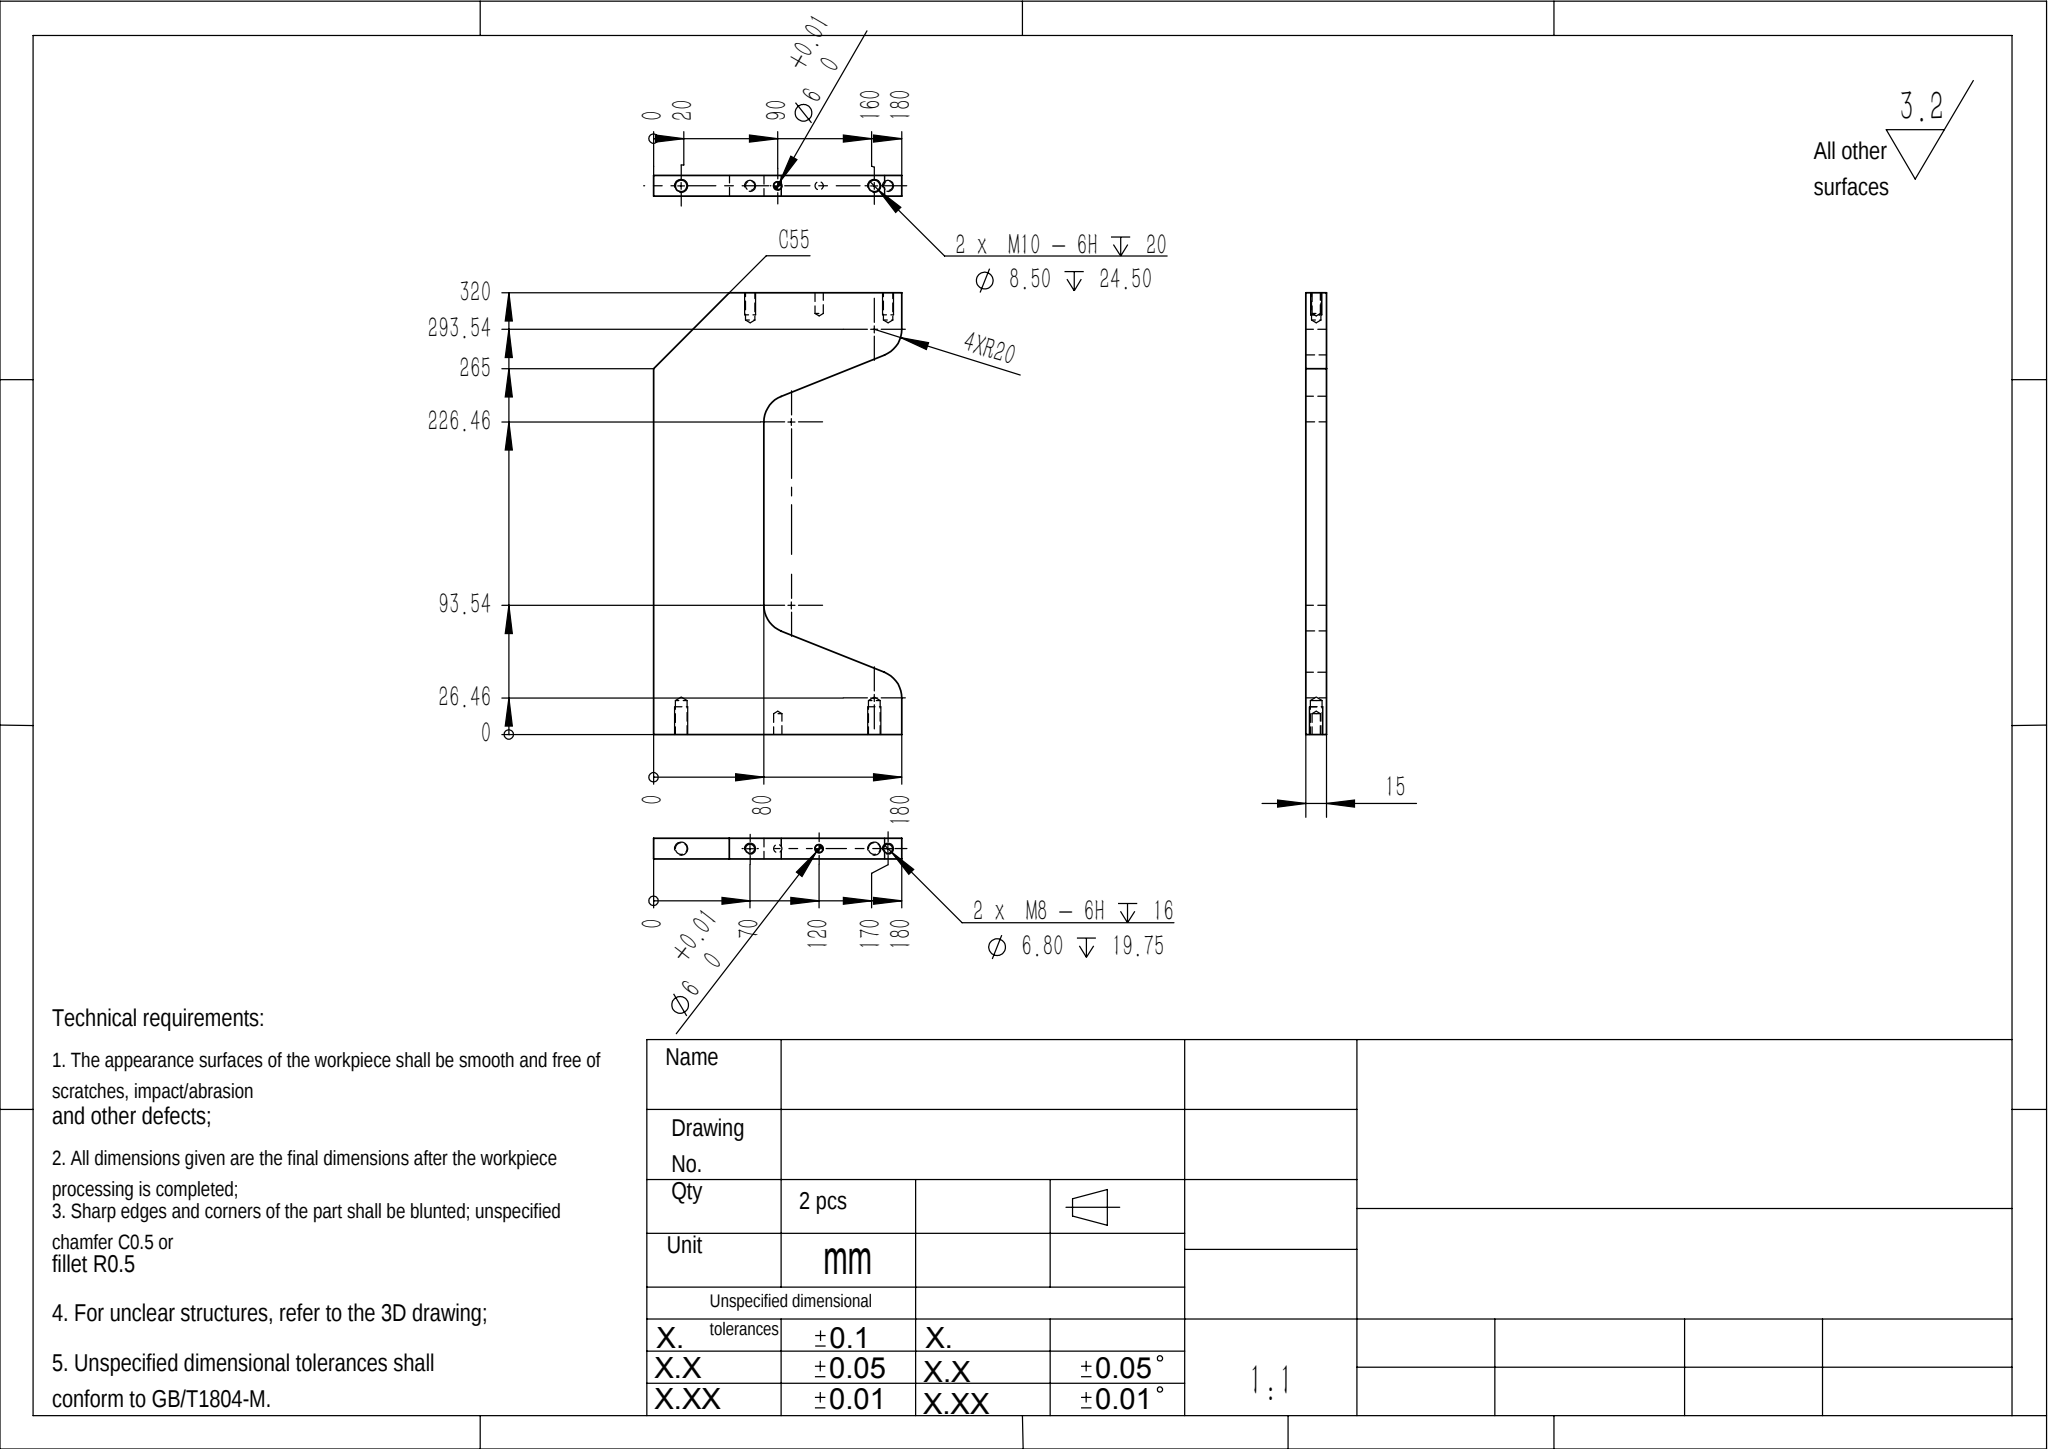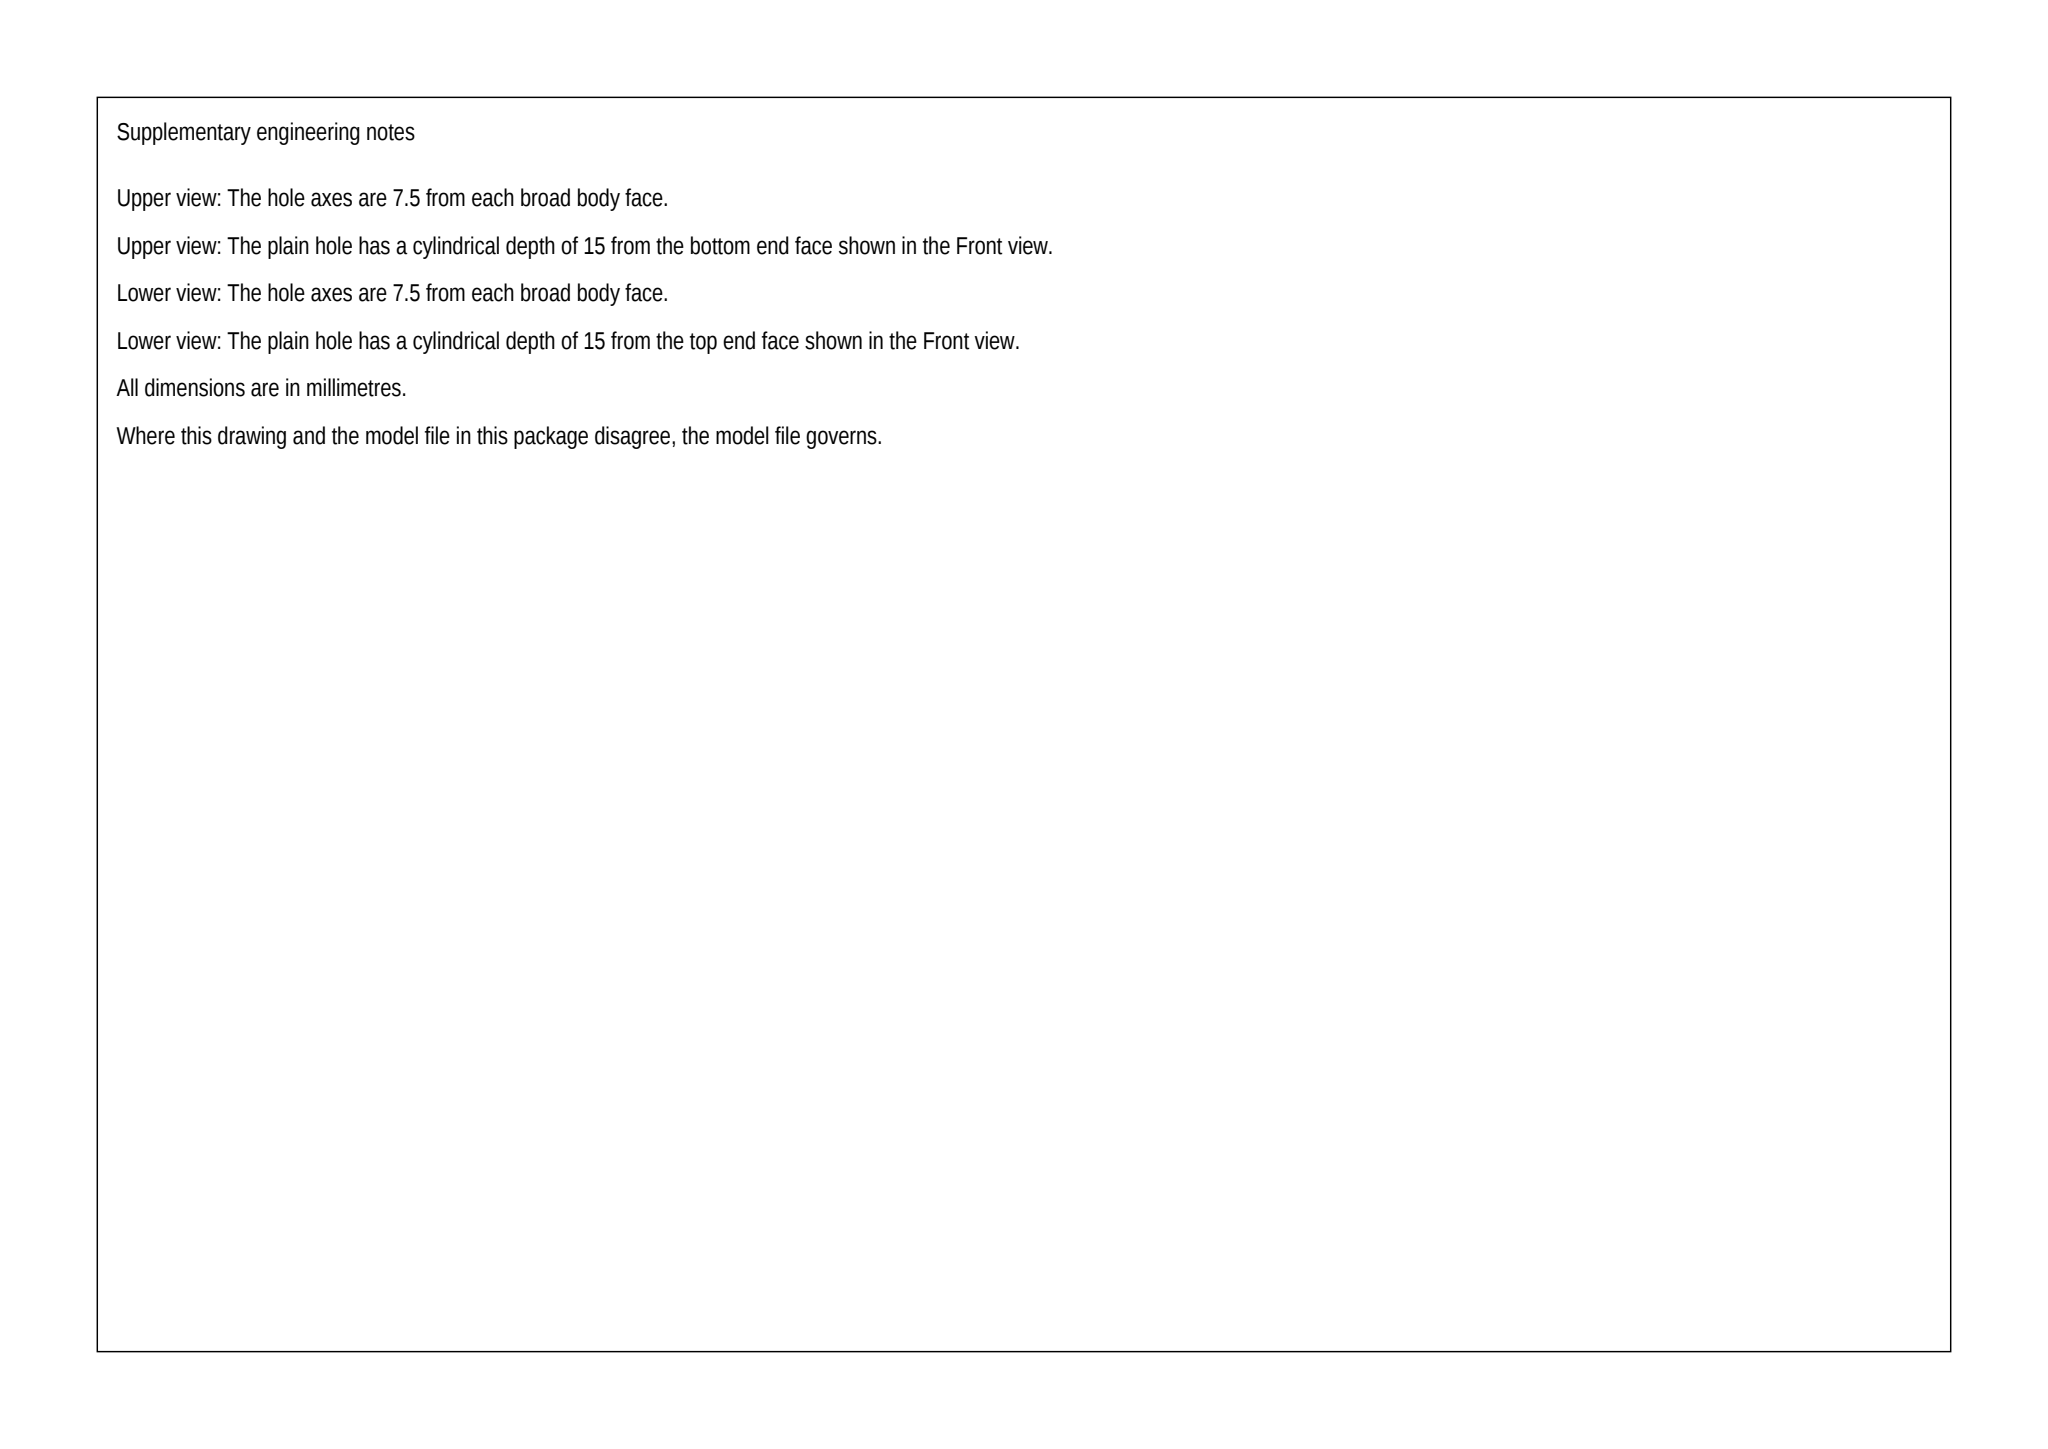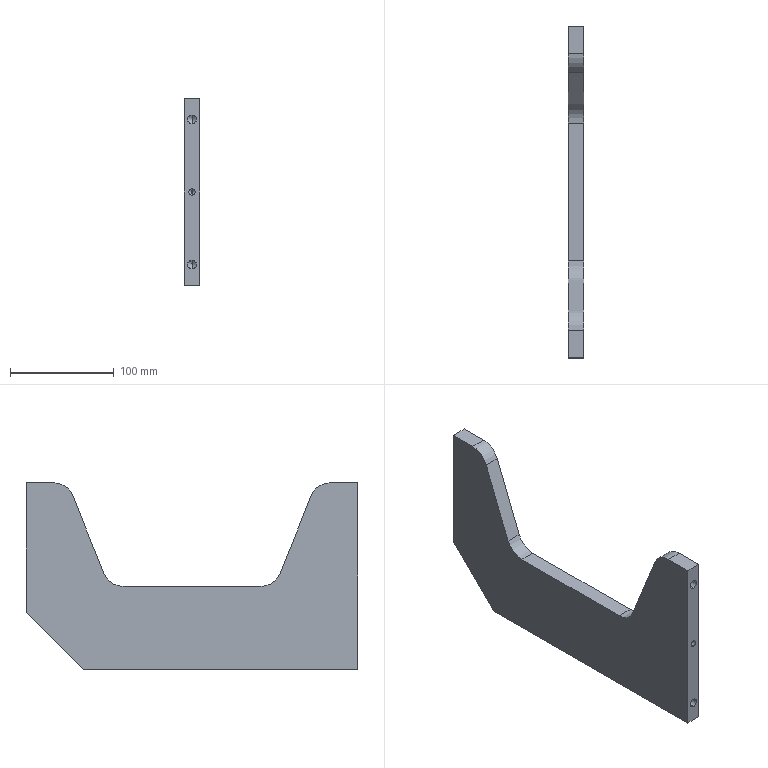Part | SolidWorks | mm | material C55 | 1 solid | 39 faces | box 15 x 320 x 180 mm | volume 536069 mm3 | cylinder 16 | cone 12 | plane 11 | commonest cylinder face diameters 6 x4 8.5 x4 6.8 x4 40 x4
build123d program:
from build123d import *

# Parameters (mm, degrees)
BOSS_EXTRUDE1_DEPTH            = 15
CHAMFER1_SIZE                  = 55
M8_TAPPED_HOLE2_D              = 6.8
M8_TAPPED_HOLE2_DEPTH          = 19.75
M8_TAPPED_HOLE2_TIP            = 2.043
M10_TAPPED_HOLE4_D             = 8.5
M10_TAPPED_HOLE4_DEPTH         = 24.5
M10_TAPPED_HOLE4_TIP           = 2.554
FILLET1_R                      = 20
SIZE_MM_DOWEL_PIN_HOLE_1_D     = 6
SIZE_MM_DOWEL_PIN_HOLE_1_DEPTH = 15
SIZE_MM_DOWEL_PIN_HOLE_1_TIP   = 1.803
SIZE_MM_DOWEL_PIN_HOLE_2_D     = 6
SIZE_MM_DOWEL_PIN_HOLE_2_DEPTH = 15
SIZE_MM_DOWEL_PIN_HOLE_2_TIP   = 1.803


with BuildPart() as part:
    # Sketch1 → Boss-Extrude1 (new body)
    with BuildSketch(Plane(origin=(0, 0, 0), x_dir=(0, 0, -1), z_dir=(1, 0, 0))):
        Polygon((0, 0), (0, 320), (-180, 320), (-180, 280), (-80, 240), (-80, 80), (-180, 40), (-180, 0), align=None)
    extrude(amount=BOSS_EXTRUDE1_DEPTH)

    # Chamfer1
    chamfer1_edges = [part.edges().sort_by_distance(p)[0] for p in [
        (7.5, 320, 0),
    ]]
    chamfer(chamfer1_edges, length=CHAMFER1_SIZE)

    # M8 Tapped Hole2
    with Locations(Plane(origin=(7.5, 320, 170), x_dir=(0, 0, 1), z_dir=(0, 1, 0))):
        with Locations((0, 0), (-100, 0)):
            Hole(M8_TAPPED_HOLE2_D / 2, depth=M8_TAPPED_HOLE2_DEPTH)
            with Locations((0, 0, -(M8_TAPPED_HOLE2_DEPTH + M8_TAPPED_HOLE2_TIP / 2))):  # 118° drill point
                Cone(0, M8_TAPPED_HOLE2_D / 2, M8_TAPPED_HOLE2_TIP, mode=Mode.SUBTRACT)

    # M10 Tapped Hole4
    with Locations(Plane(origin=(7.5, 0, 160), x_dir=(0, 0, -1), z_dir=(0, -1, 0))):
        with Locations((0, 0), (140, 0)):
            Hole(M10_TAPPED_HOLE4_D / 2, depth=M10_TAPPED_HOLE4_DEPTH)
            with Locations((0, 0, -(M10_TAPPED_HOLE4_DEPTH + M10_TAPPED_HOLE4_TIP / 2))):  # 118° drill point
                Cone(0, M10_TAPPED_HOLE4_D / 2, M10_TAPPED_HOLE4_TIP, mode=Mode.SUBTRACT)

    # Fillet1
    fillet1_edges = [part.edges().sort_by_distance(p)[0] for p in [
        (7.5, 40, 180),
        (7.5, 80, 80),
        (7.5, 240, 80),
        (7.5, 280, 180),
    ]]
    fillet(fillet1_edges, radius=FILLET1_R)

    # Size mm Dowel Pin Hole 1
    with Locations(Plane(origin=(7.5, 0, 90), x_dir=(0, 0, -1), z_dir=(0, -1, 0))):
        with Locations((0, 0)):
            Hole(SIZE_MM_DOWEL_PIN_HOLE_1_D / 2, depth=SIZE_MM_DOWEL_PIN_HOLE_1_DEPTH)
            with Locations((0, 0, -(SIZE_MM_DOWEL_PIN_HOLE_1_DEPTH + SIZE_MM_DOWEL_PIN_HOLE_1_TIP / 2))):  # 118° drill point
                Cone(0, SIZE_MM_DOWEL_PIN_HOLE_1_D / 2, SIZE_MM_DOWEL_PIN_HOLE_1_TIP, mode=Mode.SUBTRACT)

    # Size mm Dowel Pin Hole 2
    with Locations(Plane(origin=(7.5, 320, 120), x_dir=(0, 0, 1), z_dir=(0, 1, 0))):
        with Locations((0, 0)):
            Hole(SIZE_MM_DOWEL_PIN_HOLE_2_D / 2, depth=SIZE_MM_DOWEL_PIN_HOLE_2_DEPTH)
            with Locations((0, 0, -(SIZE_MM_DOWEL_PIN_HOLE_2_DEPTH + SIZE_MM_DOWEL_PIN_HOLE_2_TIP / 2))):  # 118° drill point
                Cone(0, SIZE_MM_DOWEL_PIN_HOLE_2_D / 2, SIZE_MM_DOWEL_PIN_HOLE_2_TIP, mode=Mode.SUBTRACT)


solid = part.part